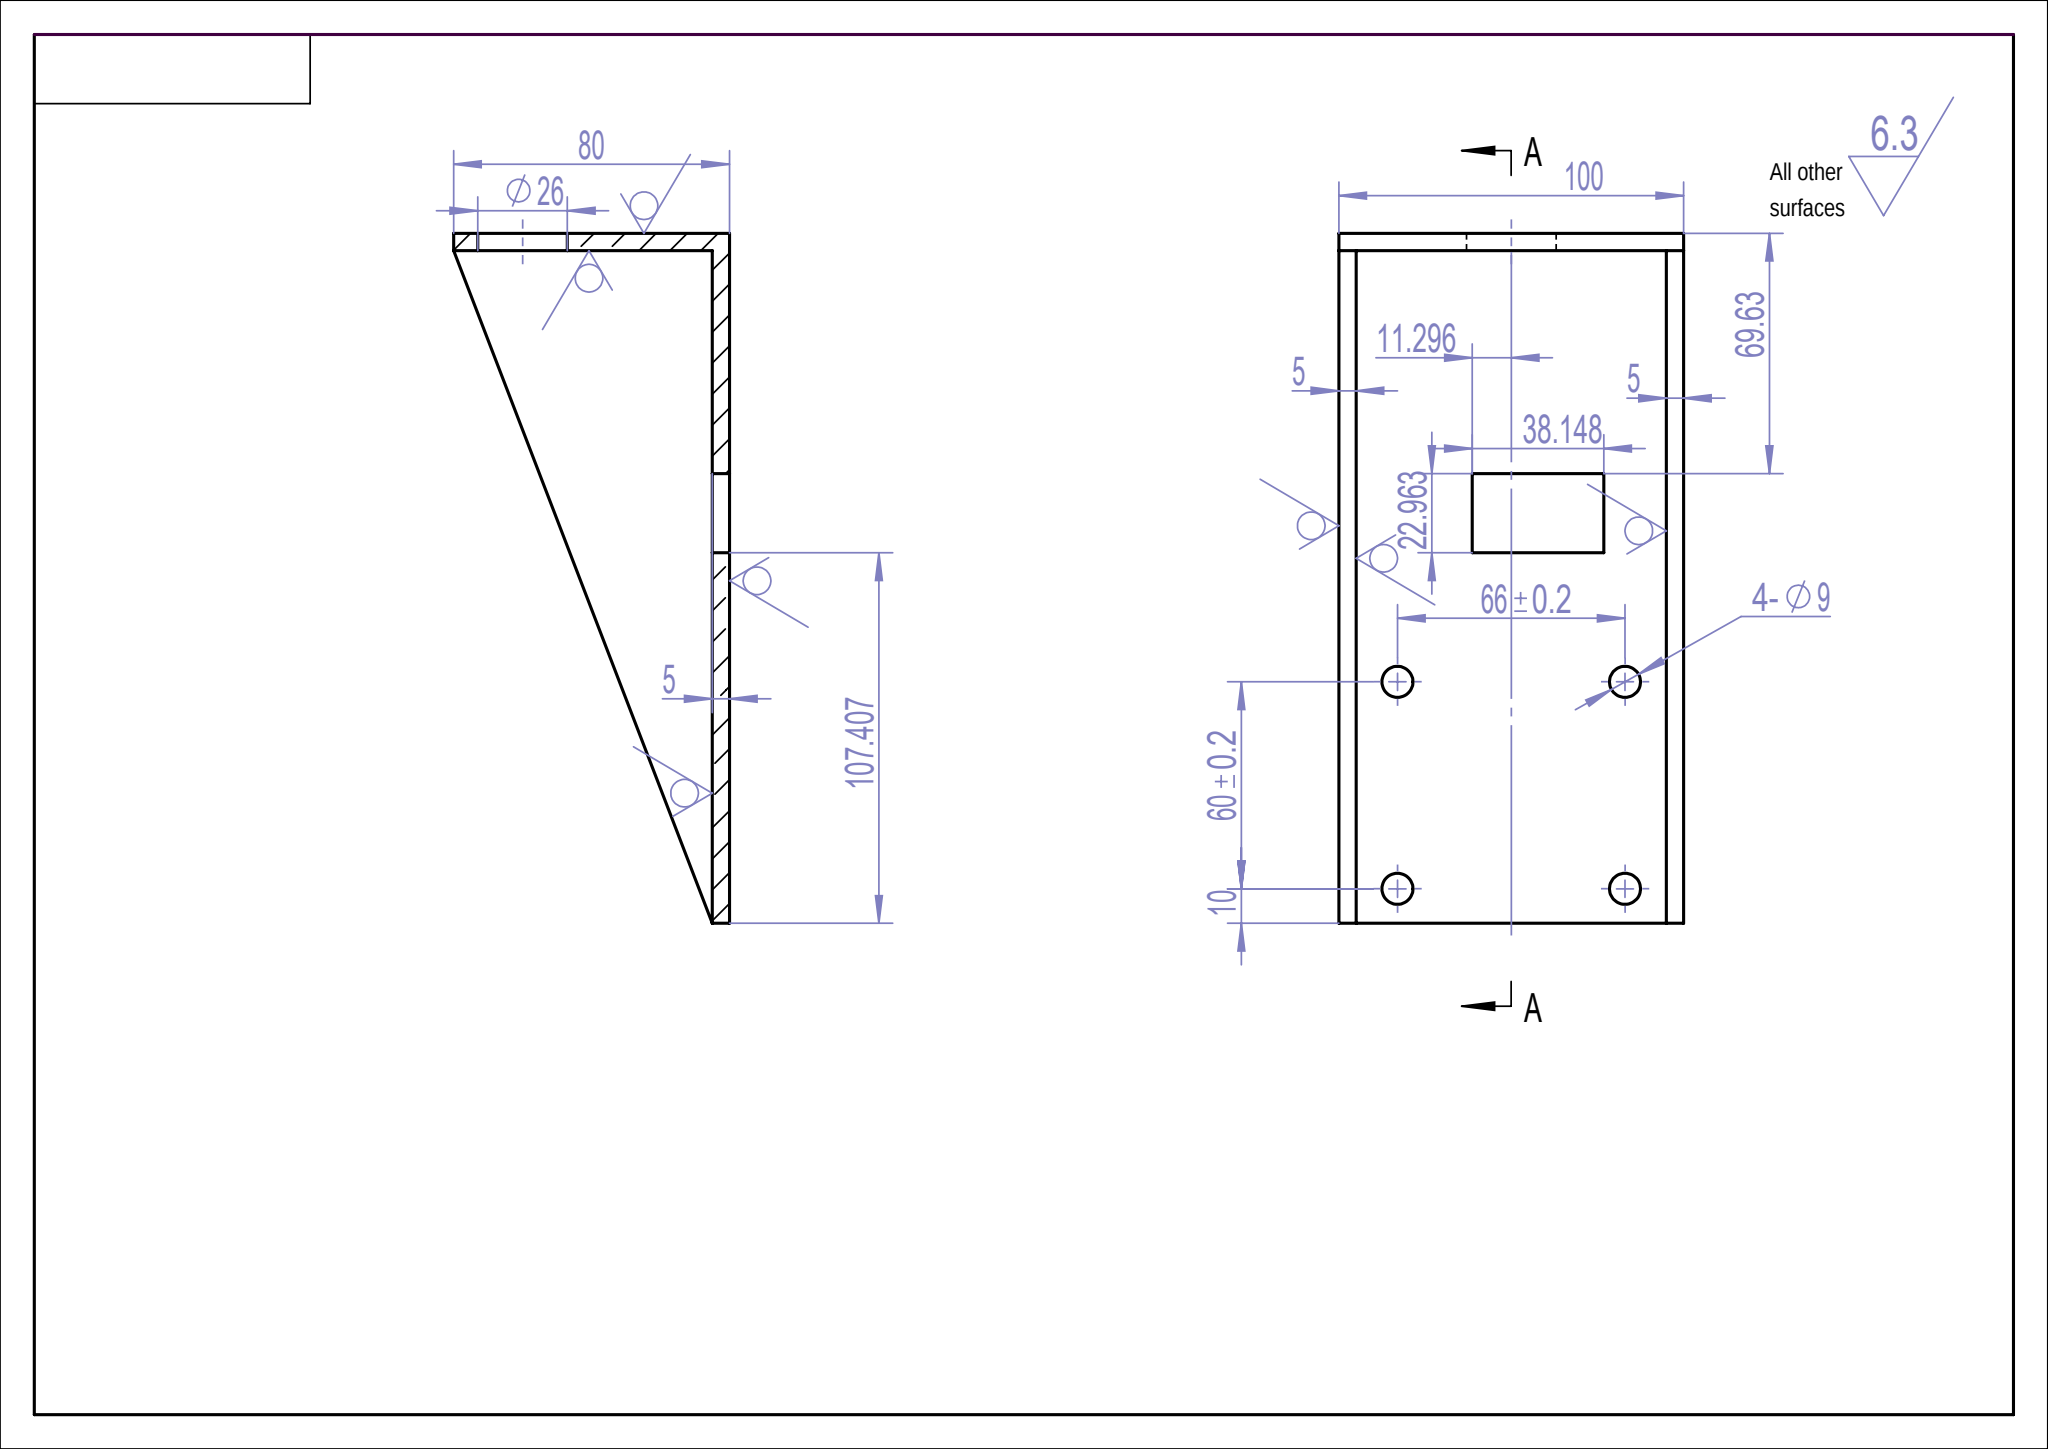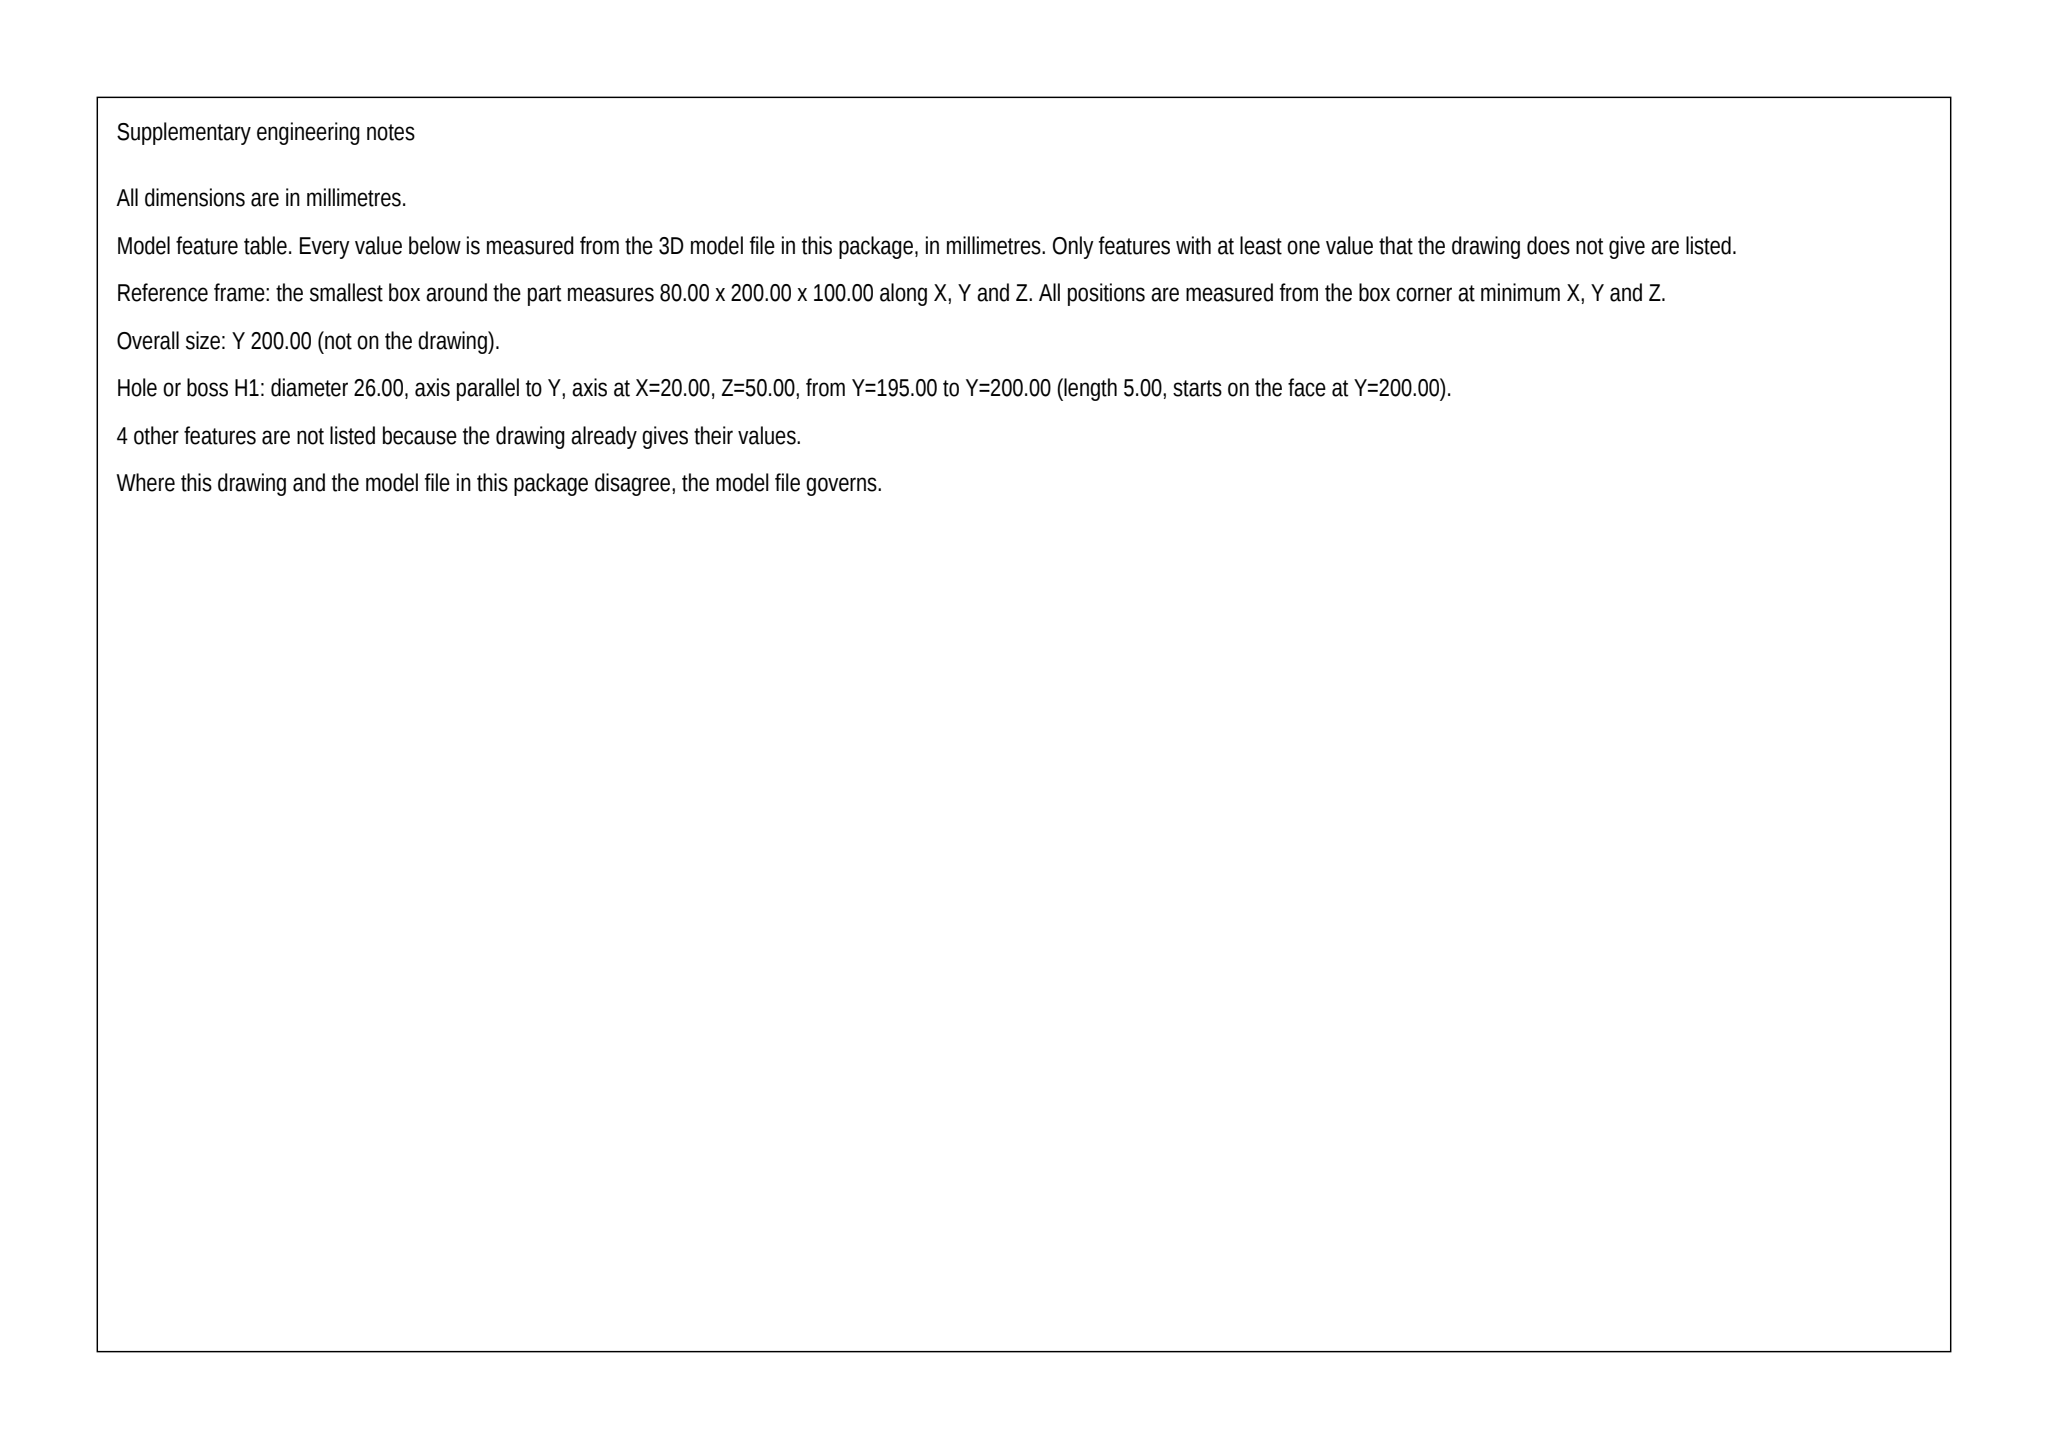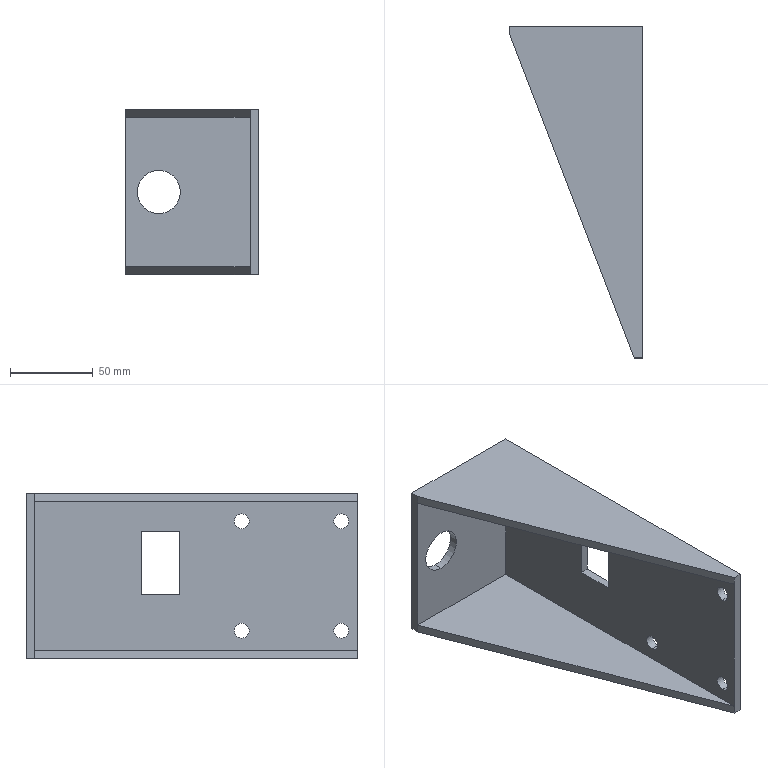Part | SolidWorks | mm | 1 solid | 26 faces | box 80 x 200 x 100 mm | volume 202318 mm3 | plane 16 | cylinder 10 | commonest cylinder face diameters 9 x8 26 x2
build123d program:
from build123d import *

# Parameters (mm, degrees)
BOSS_EXTRUDE1_DEPTH = 50
BOSS_EXTRUDE2_DEPTH = 5
SKETCH3_R           = 13
CUT_EXTRUDE1_DEPTH  = 5
SKETCH4_R           = 4.5
CUT_EXTRUDE2_DEPTH  = 5
SKETCH6_W           = 38.148
SKETCH6_H           = 22.963
CUT_EXTRUDE3_DEPTH  = 31


with BuildPart() as part:
    # Sketch1 → Boss-Extrude1 (new, symmetric)
    with BuildSketch(Plane.XY):
        Polygon((-48.173, 37.525), (31.827, 37.525), (31.827, -162.475), (26.827, -162.475), (26.827, 32.525), (-48.173, 32.525), align=None)
    extrude(amount=BOSS_EXTRUDE1_DEPTH, both=True)

    # Sketch2 → Boss-Extrude2 (add)
    with BuildSketch(Plane.XY.offset(50)):
        Polygon((-48.173, 32.525), (26.827, -162.475), (26.827, 32.525), align=None)
    boss_extrude2 = extrude(amount=-BOSS_EXTRUDE2_DEPTH)

    # Mirror1: Boss-Extrude2 across plane
    add(boss_extrude2.mirror(Plane.XY))

    # Sketch3 → Cut-Extrude1 (cut)
    with BuildSketch(Plane(origin=(0, 37.525, 0), x_dir=(1, 0, 0), z_dir=(0, 1, 0))):
        with Locations(Location((-28.173, 0, 0), (0, 0, 270))):
            Circle(SKETCH3_R)
    extrude(amount=-CUT_EXTRUDE1_DEPTH, mode=Mode.SUBTRACT)

    # Sketch4 → Cut-Extrude2 (cut)
    with BuildSketch(Plane.ZY.offset(-26.827)):
        with Locations((-33, -152.475)):
            Circle(SKETCH4_R)
        with Locations((33, -152.475)):
            Circle(SKETCH4_R)
        with Locations((-33, -92.475)):
            Circle(SKETCH4_R)
        with Locations((33, -92.475)):
            Circle(SKETCH4_R)
    extrude(amount=-CUT_EXTRUDE2_DEPTH, mode=Mode.SUBTRACT)

    # Sketch6 → Cut-Extrude3 (cut)
    with BuildSketch(Plane.ZY.offset(-26.827)):
        with Locations((7.778, -43.587)):
            Rectangle(SKETCH6_W, SKETCH6_H)
    extrude(amount=-CUT_EXTRUDE3_DEPTH, mode=Mode.SUBTRACT)


solid = part.part
STEP:
#1=CARTESIAN_POINT('',(31.827,-92.475,28.5));
#2=VERTEX_POINT('',#1);
#3=CARTESIAN_POINT('',(31.827,-92.475,37.5));
#4=VERTEX_POINT('',#3);
#5=CARTESIAN_POINT('',(31.827,-92.475,33.));
#6=DIRECTION('',(-1.,0.,0.));
#7=DIRECTION('',(0.,0.,1.));
#8=AXIS2_PLACEMENT_3D('',#5,#6,#7);
#9=CIRCLE('',#8,4.5);
#10=EDGE_CURVE('',#2,#4,#9,.T.);
#11=ORIENTED_EDGE('',*,*,#10,.F.);
#12=CARTESIAN_POINT('',(26.827,-92.475,28.5));
#13=VERTEX_POINT('',#12);
#14=CARTESIAN_POINT('',(31.827,-92.475,28.5));
#15=DIRECTION('',(-1.,0.,0.));
#16=VECTOR('',#15,1000.);
#17=LINE('',#14,#16);
#18=EDGE_CURVE('',#2,#13,#17,.T.);
#19=ORIENTED_EDGE('',*,*,#18,.T.);
#20=CARTESIAN_POINT('',(26.827,-92.475,37.5));
#21=VERTEX_POINT('',#20);
#22=CARTESIAN_POINT('',(26.827,-92.475,33.));
#23=DIRECTION('',(-1.,0.,0.));
#24=DIRECTION('',(0.,0.,1.));
#25=AXIS2_PLACEMENT_3D('',#22,#23,#24);
#26=CIRCLE('',#25,4.5);
#27=EDGE_CURVE('',#13,#21,#26,.T.);
#28=ORIENTED_EDGE('',*,*,#27,.T.);
#29=CARTESIAN_POINT('',(31.827,-92.475,37.5));
#30=DIRECTION('',(-1.,0.,0.));
#31=VECTOR('',#30,1000.);
#32=LINE('',#29,#31);
#33=EDGE_CURVE('',#4,#21,#32,.T.);
#34=ORIENTED_EDGE('',*,*,#33,.F.);
#35=EDGE_LOOP('',(#11,#19,#28,#34));
#36=FACE_OUTER_BOUND('',#35,.T.);
#37=CARTESIAN_POINT('',(31.827,-92.475,33.));
#38=DIRECTION('',(-1.,0.,0.));
#39=DIRECTION('',(0.,0.,1.));
#40=AXIS2_PLACEMENT_3D('',#37,#38,#39);
#41=CYLINDRICAL_SURFACE('',#40,4.5);
#42=ADVANCED_FACE('',(#36),#41,.F.);
#43=CARTESIAN_POINT('',(31.827,-92.475,-37.5));
#44=VERTEX_POINT('',#43);
#45=CARTESIAN_POINT('',(31.827,-92.475,-28.5));
#46=VERTEX_POINT('',#45);
#47=CARTESIAN_POINT('',(31.827,-92.475,-33.));
#48=DIRECTION('',(-1.,0.,0.));
#49=DIRECTION('',(0.,0.,1.));
#50=AXIS2_PLACEMENT_3D('',#47,#48,#49);
#51=CIRCLE('',#50,4.5);
#52=EDGE_CURVE('',#44,#46,#51,.T.);
#53=ORIENTED_EDGE('',*,*,#52,.F.);
#54=CARTESIAN_POINT('',(26.827,-92.475,-37.5));
#55=VERTEX_POINT('',#54);
#56=CARTESIAN_POINT('',(31.827,-92.475,-37.5));
#57=DIRECTION('',(-1.,0.,0.));
#58=VECTOR('',#57,1000.);
#59=LINE('',#56,#58);
#60=EDGE_CURVE('',#44,#55,#59,.T.);
#61=ORIENTED_EDGE('',*,*,#60,.T.);
#62=CARTESIAN_POINT('',(26.827,-92.475,-28.5));
#63=VERTEX_POINT('',#62);
#64=CARTESIAN_POINT('',(26.827,-92.475,-33.));
#65=DIRECTION('',(-1.,0.,0.));
#66=DIRECTION('',(0.,0.,1.));
#67=AXIS2_PLACEMENT_3D('',#64,#65,#66);
#68=CIRCLE('',#67,4.5);
#69=EDGE_CURVE('',#55,#63,#68,.T.);
#70=ORIENTED_EDGE('',*,*,#69,.T.);
#71=CARTESIAN_POINT('',(31.827,-92.475,-28.5));
#72=DIRECTION('',(-1.,0.,0.));
#73=VECTOR('',#72,1000.);
#74=LINE('',#71,#73);
#75=EDGE_CURVE('',#46,#63,#74,.T.);
#76=ORIENTED_EDGE('',*,*,#75,.F.);
#77=EDGE_LOOP('',(#53,#61,#70,#76));
#78=FACE_OUTER_BOUND('',#77,.T.);
#79=CARTESIAN_POINT('',(31.827,-92.475,-33.));
#80=DIRECTION('',(-1.,0.,0.));
#81=DIRECTION('',(0.,0.,1.));
#82=AXIS2_PLACEMENT_3D('',#79,#80,#81);
#83=CYLINDRICAL_SURFACE('',#82,4.5);
#84=ADVANCED_FACE('',(#78),#83,.F.);
#85=CARTESIAN_POINT('',(31.827,-152.475,28.5));
#86=VERTEX_POINT('',#85);
#87=CARTESIAN_POINT('',(31.827,-152.475,37.5));
#88=VERTEX_POINT('',#87);
#89=CARTESIAN_POINT('',(31.827,-152.475,33.));
#90=DIRECTION('',(-1.,0.,0.));
#91=DIRECTION('',(0.,0.,1.));
#92=AXIS2_PLACEMENT_3D('',#89,#90,#91);
#93=CIRCLE('',#92,4.5);
#94=EDGE_CURVE('',#86,#88,#93,.T.);
#95=ORIENTED_EDGE('',*,*,#94,.F.);
#96=CARTESIAN_POINT('',(26.827,-152.475,28.5));
#97=VERTEX_POINT('',#96);
#98=CARTESIAN_POINT('',(31.827,-152.475,28.5));
#99=DIRECTION('',(-1.,0.,0.));
#100=VECTOR('',#99,1000.);
#101=LINE('',#98,#100);
#102=EDGE_CURVE('',#86,#97,#101,.T.);
#103=ORIENTED_EDGE('',*,*,#102,.T.);
#104=CARTESIAN_POINT('',(26.827,-152.475,37.5));
#105=VERTEX_POINT('',#104);
#106=CARTESIAN_POINT('',(26.827,-152.475,33.));
#107=DIRECTION('',(-1.,0.,0.));
#108=DIRECTION('',(0.,0.,1.));
#109=AXIS2_PLACEMENT_3D('',#106,#107,#108);
#110=CIRCLE('',#109,4.5);
#111=EDGE_CURVE('',#97,#105,#110,.T.);
#112=ORIENTED_EDGE('',*,*,#111,.T.);
#113=CARTESIAN_POINT('',(31.827,-152.475,37.5));
#114=DIRECTION('',(-1.,0.,0.));
#115=VECTOR('',#114,1000.);
#116=LINE('',#113,#115);
#117=EDGE_CURVE('',#88,#105,#116,.T.);
#118=ORIENTED_EDGE('',*,*,#117,.F.);
#119=EDGE_LOOP('',(#95,#103,#112,#118));
#120=FACE_OUTER_BOUND('',#119,.T.);
#121=CARTESIAN_POINT('',(31.827,-152.475,33.));
#122=DIRECTION('',(-1.,0.,0.));
#123=DIRECTION('',(0.,0.,1.));
#124=AXIS2_PLACEMENT_3D('',#121,#122,#123);
#125=CYLINDRICAL_SURFACE('',#124,4.5);
#126=ADVANCED_FACE('',(#120),#125,.F.);
#127=CARTESIAN_POINT('',(31.827,-152.475,-37.5));
#128=VERTEX_POINT('',#127);
#129=CARTESIAN_POINT('',(31.827,-152.475,-28.5));
#130=VERTEX_POINT('',#129);
#131=CARTESIAN_POINT('',(31.827,-152.475,-33.));
#132=DIRECTION('',(-1.,0.,0.));
#133=DIRECTION('',(0.,0.,1.));
#134=AXIS2_PLACEMENT_3D('',#131,#132,#133);
#135=CIRCLE('',#134,4.5);
#136=EDGE_CURVE('',#128,#130,#135,.T.);
#137=ORIENTED_EDGE('',*,*,#136,.F.);
#138=CARTESIAN_POINT('',(26.827,-152.475,-37.5));
#139=VERTEX_POINT('',#138);
#140=CARTESIAN_POINT('',(31.827,-152.475,-37.5));
#141=DIRECTION('',(-1.,0.,0.));
#142=VECTOR('',#141,1000.);
#143=LINE('',#140,#142);
#144=EDGE_CURVE('',#128,#139,#143,.T.);
#145=ORIENTED_EDGE('',*,*,#144,.T.);
#146=CARTESIAN_POINT('',(26.827,-152.475,-28.5));
#147=VERTEX_POINT('',#146);
#148=CARTESIAN_POINT('',(26.827,-152.475,-33.));
#149=DIRECTION('',(-1.,0.,0.));
#150=DIRECTION('',(0.,0.,1.));
#151=AXIS2_PLACEMENT_3D('',#148,#149,#150);
#152=CIRCLE('',#151,4.5);
#153=EDGE_CURVE('',#139,#147,#152,.T.);
#154=ORIENTED_EDGE('',*,*,#153,.T.);
#155=CARTESIAN_POINT('',(31.827,-152.475,-28.5));
#156=DIRECTION('',(-1.,0.,0.));
#157=VECTOR('',#156,1000.);
#158=LINE('',#155,#157);
#159=EDGE_CURVE('',#130,#147,#158,.T.);
#160=ORIENTED_EDGE('',*,*,#159,.F.);
#161=EDGE_LOOP('',(#137,#145,#154,#160));
#162=FACE_OUTER_BOUND('',#161,.T.);
#163=CARTESIAN_POINT('',(31.827,-152.475,-33.));
#164=DIRECTION('',(-1.,0.,0.));
#165=DIRECTION('',(0.,0.,1.));
#166=AXIS2_PLACEMENT_3D('',#163,#164,#165);
#167=CYLINDRICAL_SURFACE('',#166,4.5);
#168=ADVANCED_FACE('',(#162),#167,.F.);
#169=CARTESIAN_POINT('',(-28.173,32.525,-13.));
#170=VERTEX_POINT('',#169);
#171=CARTESIAN_POINT('',(-28.173,32.525,13.));
#172=VERTEX_POINT('',#171);
#173=CARTESIAN_POINT('',(-28.173,32.525,0.));
#174=DIRECTION('',(0.,1.,0.));
#175=DIRECTION('',(0.,0.,1.));
#176=AXIS2_PLACEMENT_3D('',#173,#174,#175);
#177=CIRCLE('',#176,13.);
#178=EDGE_CURVE('',#170,#172,#177,.T.);
#179=ORIENTED_EDGE('',*,*,#178,.F.);
#180=CARTESIAN_POINT('',(-28.173,37.525,-13.));
#181=VERTEX_POINT('',#180);
#182=CARTESIAN_POINT('',(-28.173,32.525,-13.));
#183=DIRECTION('',(0.,1.,0.));
#184=VECTOR('',#183,1000.);
#185=LINE('',#182,#184);
#186=EDGE_CURVE('',#170,#181,#185,.T.);
#187=ORIENTED_EDGE('',*,*,#186,.T.);
#188=CARTESIAN_POINT('',(-28.173,37.525,13.));
#189=VERTEX_POINT('',#188);
#190=CARTESIAN_POINT('',(-28.173,37.525,0.));
#191=DIRECTION('',(0.,1.,0.));
#192=DIRECTION('',(0.,0.,1.));
#193=AXIS2_PLACEMENT_3D('',#190,#191,#192);
#194=CIRCLE('',#193,13.);
#195=EDGE_CURVE('',#181,#189,#194,.T.);
#196=ORIENTED_EDGE('',*,*,#195,.T.);
#197=CARTESIAN_POINT('',(-28.173,32.525,13.));
#198=DIRECTION('',(0.,1.,0.));
#199=VECTOR('',#198,1000.);
#200=LINE('',#197,#199);
#201=EDGE_CURVE('',#172,#189,#200,.T.);
#202=ORIENTED_EDGE('',*,*,#201,.F.);
#203=EDGE_LOOP('',(#179,#187,#196,#202));
#204=FACE_OUTER_BOUND('',#203,.T.);
#205=CARTESIAN_POINT('',(-28.173,32.525,0.));
#206=DIRECTION('',(0.,1.,0.));
#207=DIRECTION('',(0.,0.,1.));
#208=AXIS2_PLACEMENT_3D('',#205,#206,#207);
#209=CYLINDRICAL_SURFACE('',#208,13.);
#210=ADVANCED_FACE('',(#204),#209,.F.);
#211=CARTESIAN_POINT('',(-48.173,37.525,-50.));
#212=VERTEX_POINT('',#211);
#213=CARTESIAN_POINT('',(-48.173,32.525,-50.));
#214=VERTEX_POINT('',#213);
#215=CARTESIAN_POINT('',(-48.173,37.525,-50.));
#216=DIRECTION('',(0.,-1.,0.));
#217=VECTOR('',#216,1000.);
#218=LINE('',#215,#217);
#219=EDGE_CURVE('',#212,#214,#218,.T.);
#220=ORIENTED_EDGE('',*,*,#219,.T.);
#221=CARTESIAN_POINT('',(-48.173,32.525,-45.));
#222=VERTEX_POINT('',#221);
#223=CARTESIAN_POINT('',(-48.173,32.525,-45.));
#224=DIRECTION('',(0.,0.,-1.));
#225=VECTOR('',#224,1000.);
#226=LINE('',#223,#225);
#227=EDGE_CURVE('',#222,#214,#226,.T.);
#228=ORIENTED_EDGE('',*,*,#227,.F.);
#229=CARTESIAN_POINT('',(-48.173,32.525,45.));
#230=VERTEX_POINT('',#229);
#231=CARTESIAN_POINT('',(-48.173,32.525,50.));
#232=DIRECTION('',(0.,0.,-1.));
#233=VECTOR('',#232,1000.);
#234=LINE('',#231,#233);
#235=EDGE_CURVE('',#230,#222,#234,.T.);
#236=ORIENTED_EDGE('',*,*,#235,.F.);
#237=CARTESIAN_POINT('',(-48.173,32.525,50.));
#238=VERTEX_POINT('',#237);
#239=CARTESIAN_POINT('',(-48.173,32.525,50.));
#240=DIRECTION('',(0.,0.,-1.));
#241=VECTOR('',#240,1000.);
#242=LINE('',#239,#241);
#243=EDGE_CURVE('',#238,#230,#242,.T.);
#244=ORIENTED_EDGE('',*,*,#243,.F.);
#245=CARTESIAN_POINT('',(-48.173,37.525,50.));
#246=VERTEX_POINT('',#245);
#247=CARTESIAN_POINT('',(-48.173,37.525,50.));
#248=DIRECTION('',(0.,-1.,0.));
#249=VECTOR('',#248,1000.);
#250=LINE('',#247,#249);
#251=EDGE_CURVE('',#246,#238,#250,.T.);
#252=ORIENTED_EDGE('',*,*,#251,.F.);
#253=CARTESIAN_POINT('',(-48.173,37.525,50.));
#254=DIRECTION('',(0.,0.,-1.));
#255=VECTOR('',#254,1000.);
#256=LINE('',#253,#255);
#257=EDGE_CURVE('',#246,#212,#256,.T.);
#258=ORIENTED_EDGE('',*,*,#257,.T.);
#259=EDGE_LOOP('',(#220,#228,#236,#244,#252,#258));
#260=FACE_OUTER_BOUND('',#259,.T.);
#261=CARTESIAN_POINT('',(-48.173,37.525,50.));
#262=DIRECTION('',(1.,0.,0.));
#263=DIRECTION('',(0.,0.,-1.));
#264=AXIS2_PLACEMENT_3D('',#261,#262,#263);
#265=PLANE('',#264);
#266=ADVANCED_FACE('',(#260),#265,.F.);
#267=CARTESIAN_POINT('',(-28.173,32.525,0.));
#268=DIRECTION('',(0.,1.,0.));
#269=DIRECTION('',(0.,0.,1.));
#270=AXIS2_PLACEMENT_3D('',#267,#268,#269);
#271=CIRCLE('',#270,13.);
#272=EDGE_CURVE('',#172,#170,#271,.T.);
#273=ORIENTED_EDGE('',*,*,#272,.T.);
#274=ORIENTED_EDGE('',*,*,#178,.T.);
#275=EDGE_LOOP('',(#273,#274));
#276=FACE_BOUND('',#275,.T.);
#277=ORIENTED_EDGE('',*,*,#235,.T.);
#278=CARTESIAN_POINT('',(26.827,32.525,-45.));
#279=VERTEX_POINT('',#278);
#280=CARTESIAN_POINT('',(26.827,32.525,-45.));
#281=DIRECTION('',(-1.,0.,0.));
#282=VECTOR('',#281,1000.);
#283=LINE('',#280,#282);
#284=EDGE_CURVE('',#279,#222,#283,.T.);
#285=ORIENTED_EDGE('',*,*,#284,.F.);
#286=CARTESIAN_POINT('',(26.827,32.525,45.));
#287=VERTEX_POINT('',#286);
#288=CARTESIAN_POINT('',(26.827,32.525,50.));
#289=DIRECTION('',(0.,0.,-1.));
#290=VECTOR('',#289,1000.);
#291=LINE('',#288,#290);
#292=EDGE_CURVE('',#287,#279,#291,.T.);
#293=ORIENTED_EDGE('',*,*,#292,.F.);
#294=CARTESIAN_POINT('',(26.827,32.525,45.));
#295=DIRECTION('',(-1.,0.,0.));
#296=VECTOR('',#295,1000.);
#297=LINE('',#294,#296);
#298=EDGE_CURVE('',#287,#230,#297,.T.);
#299=ORIENTED_EDGE('',*,*,#298,.T.);
#300=EDGE_LOOP('',(#277,#285,#293,#299));
#301=FACE_OUTER_BOUND('',#300,.T.);
#302=CARTESIAN_POINT('',(-48.173,32.525,50.));
#303=DIRECTION('',(0.,1.,0.));
#304=DIRECTION('',(0.,0.,1.));
#305=AXIS2_PLACEMENT_3D('',#302,#303,#304);
#306=PLANE('',#305);
#307=ADVANCED_FACE('',(#276,#301),#306,.F.);
#308=CARTESIAN_POINT('',(26.827,-55.068,-11.296));
#309=VERTEX_POINT('',#308);
#310=CARTESIAN_POINT('',(26.827,-55.068,26.852));
#311=VERTEX_POINT('',#310);
#312=CARTESIAN_POINT('',(26.827,-55.068,-11.296));
#313=DIRECTION('',(0.,0.,1.));
#314=VECTOR('',#313,1000.);
#315=LINE('',#312,#314);
#316=EDGE_CURVE('',#309,#311,#315,.T.);
#317=ORIENTED_EDGE('',*,*,#316,.F.);
#318=CARTESIAN_POINT('',(26.827,-32.105,-11.296));
#319=VERTEX_POINT('',#318);
#320=CARTESIAN_POINT('',(26.827,-32.105,-11.296));
#321=DIRECTION('',(0.,-1.,0.));
#322=VECTOR('',#321,1000.);
#323=LINE('',#320,#322);
#324=EDGE_CURVE('',#319,#309,#323,.T.);
#325=ORIENTED_EDGE('',*,*,#324,.F.);
#326=CARTESIAN_POINT('',(26.827,-32.105,26.852));
#327=VERTEX_POINT('',#326);
#328=CARTESIAN_POINT('',(26.827,-32.105,-11.296));
#329=DIRECTION('',(0.,0.,-1.));
#330=VECTOR('',#329,1000.);
#331=LINE('',#328,#330);
#332=EDGE_CURVE('',#327,#319,#331,.T.);
#333=ORIENTED_EDGE('',*,*,#332,.F.);
#334=CARTESIAN_POINT('',(26.827,-32.105,26.852));
#335=DIRECTION('',(0.,1.,0.));
#336=VECTOR('',#335,1000.);
#337=LINE('',#334,#336);
#338=EDGE_CURVE('',#311,#327,#337,.T.);
#339=ORIENTED_EDGE('',*,*,#338,.F.);
#340=EDGE_LOOP('',(#317,#325,#333,#339));
#341=FACE_BOUND('',#340,.T.);
#342=CARTESIAN_POINT('',(26.827,-92.475,33.));
#343=DIRECTION('',(-1.,0.,0.));
#344=DIRECTION('',(0.,0.,1.));
#345=AXIS2_PLACEMENT_3D('',#342,#343,#344);
#346=CIRCLE('',#345,4.5);
#347=EDGE_CURVE('',#21,#13,#346,.T.);
#348=ORIENTED_EDGE('',*,*,#347,.F.);
#349=ORIENTED_EDGE('',*,*,#27,.F.);
#350=EDGE_LOOP('',(#348,#349));
#351=FACE_BOUND('',#350,.T.);
#352=CARTESIAN_POINT('',(26.827,-92.475,-33.));
#353=DIRECTION('',(-1.,0.,0.));
#354=DIRECTION('',(0.,0.,1.));
#355=AXIS2_PLACEMENT_3D('',#352,#353,#354);
#356=CIRCLE('',#355,4.5);
#357=EDGE_CURVE('',#63,#55,#356,.T.);
#358=ORIENTED_EDGE('',*,*,#357,.F.);
#359=ORIENTED_EDGE('',*,*,#69,.F.);
#360=EDGE_LOOP('',(#358,#359));
#361=FACE_BOUND('',#360,.T.);
#362=CARTESIAN_POINT('',(26.827,-152.475,33.));
#363=DIRECTION('',(-1.,0.,0.));
#364=DIRECTION('',(0.,0.,1.));
#365=AXIS2_PLACEMENT_3D('',#362,#363,#364);
#366=CIRCLE('',#365,4.5);
#367=EDGE_CURVE('',#105,#97,#366,.T.);
#368=ORIENTED_EDGE('',*,*,#367,.F.);
#369=ORIENTED_EDGE('',*,*,#111,.F.);
#370=EDGE_LOOP('',(#368,#369));
#371=FACE_BOUND('',#370,.T.);
#372=CARTESIAN_POINT('',(26.827,-152.475,-33.));
#373=DIRECTION('',(-1.,0.,0.));
#374=DIRECTION('',(0.,0.,1.));
#375=AXIS2_PLACEMENT_3D('',#372,#373,#374);
#376=CIRCLE('',#375,4.5);
#377=EDGE_CURVE('',#147,#139,#376,.T.);
#378=ORIENTED_EDGE('',*,*,#377,.F.);
#379=ORIENTED_EDGE('',*,*,#153,.F.);
#380=EDGE_LOOP('',(#378,#379));
#381=FACE_BOUND('',#380,.T.);
#382=ORIENTED_EDGE('',*,*,#292,.T.);
#383=CARTESIAN_POINT('',(26.827,-162.475,-45.));
#384=VERTEX_POINT('',#383);
#385=CARTESIAN_POINT('',(26.827,-162.475,-45.));
#386=DIRECTION('',(0.,1.,0.));
#387=VECTOR('',#386,1000.);
#388=LINE('',#385,#387);
#389=EDGE_CURVE('',#384,#279,#388,.T.);
#390=ORIENTED_EDGE('',*,*,#389,.F.);
#391=CARTESIAN_POINT('',(26.827,-162.475,45.));
#392=VERTEX_POINT('',#391);
#393=CARTESIAN_POINT('',(26.827,-162.475,50.));
#394=DIRECTION('',(0.,0.,-1.));
#395=VECTOR('',#394,1000.);
#396=LINE('',#393,#395);
#397=EDGE_CURVE('',#392,#384,#396,.T.);
#398=ORIENTED_EDGE('',*,*,#397,.F.);
#399=CARTESIAN_POINT('',(26.827,-162.475,45.));
#400=DIRECTION('',(0.,1.,0.));
#401=VECTOR('',#400,1000.);
#402=LINE('',#399,#401);
#403=EDGE_CURVE('',#392,#287,#402,.T.);
#404=ORIENTED_EDGE('',*,*,#403,.T.);
#405=EDGE_LOOP('',(#382,#390,#398,#404));
#406=FACE_OUTER_BOUND('',#405,.T.);
#407=CARTESIAN_POINT('',(26.827,32.525,50.));
#408=DIRECTION('',(1.,0.,0.));
#409=DIRECTION('',(0.,0.,-1.));
#410=AXIS2_PLACEMENT_3D('',#407,#408,#409);
#411=PLANE('',#410);
#412=ADVANCED_FACE('',(#341,#351,#361,#371,#381,#406),#411,.F.);
#413=CARTESIAN_POINT('',(26.827,-162.475,-50.));
#414=VERTEX_POINT('',#413);
#415=CARTESIAN_POINT('',(31.827,-162.475,-50.));
#416=VERTEX_POINT('',#415);
#417=CARTESIAN_POINT('',(26.827,-162.475,-50.));
#418=DIRECTION('',(1.,0.,0.));
#419=VECTOR('',#418,1000.);
#420=LINE('',#417,#419);
#421=EDGE_CURVE('',#414,#416,#420,.T.);
#422=ORIENTED_EDGE('',*,*,#421,.T.);
#423=CARTESIAN_POINT('',(31.827,-162.475,50.));
#424=VERTEX_POINT('',#423);
#425=CARTESIAN_POINT('',(31.827,-162.475,50.));
#426=DIRECTION('',(0.,0.,-1.));
#427=VECTOR('',#426,1000.);
#428=LINE('',#425,#427);
#429=EDGE_CURVE('',#424,#416,#428,.T.);
#430=ORIENTED_EDGE('',*,*,#429,.F.);
#431=CARTESIAN_POINT('',(26.827,-162.475,50.));
#432=VERTEX_POINT('',#431);
#433=CARTESIAN_POINT('',(26.827,-162.475,50.));
#434=DIRECTION('',(1.,0.,0.));
#435=VECTOR('',#434,1000.);
#436=LINE('',#433,#435);
#437=EDGE_CURVE('',#432,#424,#436,.T.);
#438=ORIENTED_EDGE('',*,*,#437,.F.);
#439=CARTESIAN_POINT('',(26.827,-162.475,50.));
#440=DIRECTION('',(0.,0.,-1.));
#441=VECTOR('',#440,1000.);
#442=LINE('',#439,#441);
#443=EDGE_CURVE('',#432,#392,#442,.T.);
#444=ORIENTED_EDGE('',*,*,#443,.T.);
#445=ORIENTED_EDGE('',*,*,#397,.T.);
#446=CARTESIAN_POINT('',(26.827,-162.475,-45.));
#447=DIRECTION('',(0.,0.,-1.));
#448=VECTOR('',#447,1000.);
#449=LINE('',#446,#448);
#450=EDGE_CURVE('',#384,#414,#449,.T.);
#451=ORIENTED_EDGE('',*,*,#450,.T.);
#452=EDGE_LOOP('',(#422,#430,#438,#444,#445,#451));
#453=FACE_OUTER_BOUND('',#452,.T.);
#454=CARTESIAN_POINT('',(26.827,-162.475,50.));
#455=DIRECTION('',(0.,1.,0.));
#456=DIRECTION('',(0.,0.,1.));
#457=AXIS2_PLACEMENT_3D('',#454,#455,#456);
#458=PLANE('',#457);
#459=ADVANCED_FACE('',(#453),#458,.F.);
#460=CARTESIAN_POINT('',(31.827,-32.105,26.852));
#461=VERTEX_POINT('',#460);
#462=CARTESIAN_POINT('',(31.827,-32.105,-11.296));
#463=VERTEX_POINT('',#462);
#464=CARTESIAN_POINT('',(31.827,-32.105,50.));
#465=DIRECTION('',(0.,0.,-1.));
#466=VECTOR('',#465,1000.);
#467=LINE('',#464,#466);
#468=EDGE_CURVE('',#461,#463,#467,.T.);
#469=ORIENTED_EDGE('',*,*,#468,.T.);
#470=CARTESIAN_POINT('',(31.827,-55.068,-11.296));
#471=VERTEX_POINT('',#470);
#472=CARTESIAN_POINT('',(31.827,37.525,-11.296));
#473=DIRECTION('',(0.,-1.,0.));
#474=VECTOR('',#473,1000.);
#475=LINE('',#472,#474);
#476=EDGE_CURVE('',#463,#471,#475,.T.);
#477=ORIENTED_EDGE('',*,*,#476,.T.);
#478=CARTESIAN_POINT('',(31.827,-55.068,26.852));
#479=VERTEX_POINT('',#478);
#480=CARTESIAN_POINT('',(31.827,-55.068,50.));
#481=DIRECTION('',(0.,0.,1.));
#482=VECTOR('',#481,1000.);
#483=LINE('',#480,#482);
#484=EDGE_CURVE('',#471,#479,#483,.T.);
#485=ORIENTED_EDGE('',*,*,#484,.T.);
#486=CARTESIAN_POINT('',(31.827,37.525,26.852));
#487=DIRECTION('',(-0.,1.,0.));
#488=VECTOR('',#487,1000.);
#489=LINE('',#486,#488);
#490=EDGE_CURVE('',#479,#461,#489,.T.);
#491=ORIENTED_EDGE('',*,*,#490,.T.);
#492=EDGE_LOOP('',(#469,#477,#485,#491));
#493=FACE_BOUND('',#492,.T.);
#494=CARTESIAN_POINT('',(31.827,-92.475,33.));
#495=DIRECTION('',(-1.,0.,0.));
#496=DIRECTION('',(0.,0.,1.));
#497=AXIS2_PLACEMENT_3D('',#494,#495,#496);
#498=CIRCLE('',#497,4.5);
#499=EDGE_CURVE('',#4,#2,#498,.T.);
#500=ORIENTED_EDGE('',*,*,#499,.T.);
#501=ORIENTED_EDGE('',*,*,#10,.T.);
#502=EDGE_LOOP('',(#500,#501));
#503=FACE_BOUND('',#502,.T.);
#504=CARTESIAN_POINT('',(31.827,-92.475,-33.));
#505=DIRECTION('',(-1.,0.,0.));
#506=DIRECTION('',(0.,0.,1.));
#507=AXIS2_PLACEMENT_3D('',#504,#505,#506);
#508=CIRCLE('',#507,4.5);
#509=EDGE_CURVE('',#46,#44,#508,.T.);
#510=ORIENTED_EDGE('',*,*,#509,.T.);
#511=ORIENTED_EDGE('',*,*,#52,.T.);
#512=EDGE_LOOP('',(#510,#511));
#513=FACE_BOUND('',#512,.T.);
#514=CARTESIAN_POINT('',(31.827,-152.475,33.));
#515=DIRECTION('',(-1.,0.,0.));
#516=DIRECTION('',(0.,0.,1.));
#517=AXIS2_PLACEMENT_3D('',#514,#515,#516);
#518=CIRCLE('',#517,4.5);
#519=EDGE_CURVE('',#88,#86,#518,.T.);
#520=ORIENTED_EDGE('',*,*,#519,.T.);
#521=ORIENTED_EDGE('',*,*,#94,.T.);
#522=EDGE_LOOP('',(#520,#521));
#523=FACE_BOUND('',#522,.T.);
#524=CARTESIAN_POINT('',(31.827,-152.475,-33.));
#525=DIRECTION('',(-1.,0.,0.));
#526=DIRECTION('',(0.,0.,1.));
#527=AXIS2_PLACEMENT_3D('',#524,#525,#526);
#528=CIRCLE('',#527,4.5);
#529=EDGE_CURVE('',#130,#128,#528,.T.);
#530=ORIENTED_EDGE('',*,*,#529,.T.);
#531=ORIENTED_EDGE('',*,*,#136,.T.);
#532=EDGE_LOOP('',(#530,#531));
#533=FACE_BOUND('',#532,.T.);
#534=CARTESIAN_POINT('',(31.827,37.525,-50.));
#535=VERTEX_POINT('',#534);
#536=CARTESIAN_POINT('',(31.827,37.525,-50.));
#537=DIRECTION('',(-0.,1.,0.));
#538=VECTOR('',#537,1000.);
#539=LINE('',#536,#538);
#540=EDGE_CURVE('',#416,#535,#539,.T.);
#541=ORIENTED_EDGE('',*,*,#540,.T.);
#542=CARTESIAN_POINT('',(31.827,37.525,50.));
#543=VERTEX_POINT('',#542);
#544=CARTESIAN_POINT('',(31.827,37.525,50.));
#545=DIRECTION('',(0.,0.,-1.));
#546=VECTOR('',#545,1000.);
#547=LINE('',#544,#546);
#548=EDGE_CURVE('',#543,#535,#547,.T.);
#549=ORIENTED_EDGE('',*,*,#548,.F.);
#550=CARTESIAN_POINT('',(31.827,37.525,50.));
#551=DIRECTION('',(-0.,1.,0.));
#552=VECTOR('',#551,1000.);
#553=LINE('',#550,#552);
#554=EDGE_CURVE('',#424,#543,#553,.T.);
#555=ORIENTED_EDGE('',*,*,#554,.F.);
#556=ORIENTED_EDGE('',*,*,#429,.T.);
#557=EDGE_LOOP('',(#541,#549,#555,#556));
#558=FACE_OUTER_BOUND('',#557,.T.);
#559=CARTESIAN_POINT('',(31.827,37.525,50.));
#560=DIRECTION('',(-1.,-0.,0.));
#561=DIRECTION('',(0.,-1.,0.));
#562=AXIS2_PLACEMENT_3D('',#559,#560,#561);
#563=PLANE('',#562);
#564=ADVANCED_FACE('',(#493,#503,#513,#523,#533,#558),#563,.F.);
#565=CARTESIAN_POINT('',(-28.173,37.525,0.));
#566=DIRECTION('',(0.,1.,0.));
#567=DIRECTION('',(0.,0.,1.));
#568=AXIS2_PLACEMENT_3D('',#565,#566,#567);
#569=CIRCLE('',#568,13.);
#570=EDGE_CURVE('',#189,#181,#569,.T.);
#571=ORIENTED_EDGE('',*,*,#570,.F.);
#572=ORIENTED_EDGE('',*,*,#195,.F.);
#573=EDGE_LOOP('',(#571,#572));
#574=FACE_BOUND('',#573,.T.);
#575=CARTESIAN_POINT('',(-48.173,37.525,-50.));
#576=DIRECTION('',(-1.,0.,0.));
#577=VECTOR('',#576,1000.);
#578=LINE('',#575,#577);
#579=EDGE_CURVE('',#535,#212,#578,.T.);
#580=ORIENTED_EDGE('',*,*,#579,.T.);
#581=ORIENTED_EDGE('',*,*,#257,.F.);
#582=CARTESIAN_POINT('',(-48.173,37.525,50.));
#583=DIRECTION('',(-1.,0.,0.));
#584=VECTOR('',#583,1000.);
#585=LINE('',#582,#584);
#586=EDGE_CURVE('',#543,#246,#585,.T.);
#587=ORIENTED_EDGE('',*,*,#586,.F.);
#588=ORIENTED_EDGE('',*,*,#548,.T.);
#589=EDGE_LOOP('',(#580,#581,#587,#588));
#590=FACE_OUTER_BOUND('',#589,.T.);
#591=CARTESIAN_POINT('',(-48.173,37.525,50.));
#592=DIRECTION('',(0.,-1.,0.));
#593=DIRECTION('',(0.,0.,-1.));
#594=AXIS2_PLACEMENT_3D('',#591,#592,#593);
#595=PLANE('',#594);
#596=ADVANCED_FACE('',(#574,#590),#595,.F.);
#597=ORIENTED_EDGE('',*,*,#251,.T.);
#598=CARTESIAN_POINT('',(-48.173,32.525,50.));
#599=DIRECTION('',(0.359,-0.9333,0.));
#600=VECTOR('',#599,1000.);
#601=LINE('',#598,#600);
#602=EDGE_CURVE('',#238,#432,#601,.T.);
#603=ORIENTED_EDGE('',*,*,#602,.T.);
#604=ORIENTED_EDGE('',*,*,#437,.T.);
#605=ORIENTED_EDGE('',*,*,#554,.T.);
#606=ORIENTED_EDGE('',*,*,#586,.T.);
#607=EDGE_LOOP('',(#597,#603,#604,#605,#606));
#608=FACE_OUTER_BOUND('',#607,.T.);
#609=CARTESIAN_POINT('',(0.,0.,50.));
#610=DIRECTION('',(0.,0.,1.));
#611=DIRECTION('',(1.,0.,0.));
#612=AXIS2_PLACEMENT_3D('',#609,#610,#611);
#613=PLANE('',#612);
#614=ADVANCED_FACE('',(#608),#613,.T.);
#615=ORIENTED_EDGE('',*,*,#219,.F.);
#616=ORIENTED_EDGE('',*,*,#579,.F.);
#617=ORIENTED_EDGE('',*,*,#540,.F.);
#618=ORIENTED_EDGE('',*,*,#421,.F.);
#619=CARTESIAN_POINT('',(-48.173,32.525,-50.));
#620=DIRECTION('',(0.359,-0.9333,0.));
#621=VECTOR('',#620,1000.);
#622=LINE('',#619,#621);
#623=EDGE_CURVE('',#214,#414,#622,.T.);
#624=ORIENTED_EDGE('',*,*,#623,.F.);
#625=EDGE_LOOP('',(#615,#616,#617,#618,#624));
#626=FACE_OUTER_BOUND('',#625,.T.);
#627=CARTESIAN_POINT('',(0.,0.,-50.));
#628=DIRECTION('',(0.,0.,1.));
#629=DIRECTION('',(1.,0.,0.));
#630=AXIS2_PLACEMENT_3D('',#627,#628,#629);
#631=PLANE('',#630);
#632=ADVANCED_FACE('',(#626),#631,.F.);
#633=ORIENTED_EDGE('',*,*,#602,.F.);
#634=ORIENTED_EDGE('',*,*,#243,.T.);
#635=CARTESIAN_POINT('',(-48.173,32.525,45.));
#636=DIRECTION('',(0.359,-0.9333,0.));
#637=VECTOR('',#636,1000.);
#638=LINE('',#635,#637);
#639=EDGE_CURVE('',#230,#392,#638,.T.);
#640=ORIENTED_EDGE('',*,*,#639,.T.);
#641=ORIENTED_EDGE('',*,*,#443,.F.);
#642=EDGE_LOOP('',(#633,#634,#640,#641));
#643=FACE_OUTER_BOUND('',#642,.T.);
#644=CARTESIAN_POINT('',(-48.173,32.525,45.));
#645=DIRECTION('',(-0.9333,-0.359,0.));
#646=DIRECTION('',(0.359,-0.9333,0.));
#647=AXIS2_PLACEMENT_3D('',#644,#645,#646);
#648=PLANE('',#647);
#649=ADVANCED_FACE('',(#643),#648,.T.);
#650=ORIENTED_EDGE('',*,*,#298,.F.);
#651=ORIENTED_EDGE('',*,*,#403,.F.);
#652=ORIENTED_EDGE('',*,*,#639,.F.);
#653=EDGE_LOOP('',(#650,#651,#652));
#654=FACE_OUTER_BOUND('',#653,.T.);
#655=CARTESIAN_POINT('',(0.,0.,45.));
#656=DIRECTION('',(0.,0.,-1.));
#657=DIRECTION('',(-1.,0.,0.));
#658=AXIS2_PLACEMENT_3D('',#655,#656,#657);
#659=PLANE('',#658);
#660=ADVANCED_FACE('',(#654),#659,.T.);
#661=ORIENTED_EDGE('',*,*,#623,.T.);
#662=ORIENTED_EDGE('',*,*,#450,.F.);
#663=CARTESIAN_POINT('',(-48.173,32.525,-45.));
#664=DIRECTION('',(0.359,-0.9333,0.));
#665=VECTOR('',#664,1000.);
#666=LINE('',#663,#665);
#667=EDGE_CURVE('',#222,#384,#666,.T.);
#668=ORIENTED_EDGE('',*,*,#667,.F.);
#669=ORIENTED_EDGE('',*,*,#227,.T.);
#670=EDGE_LOOP('',(#661,#662,#668,#669));
#671=FACE_OUTER_BOUND('',#670,.T.);
#672=CARTESIAN_POINT('',(-48.173,32.525,-45.));
#673=DIRECTION('',(0.9333,0.359,0.));
#674=DIRECTION('',(-0.359,0.9333,0.));
#675=AXIS2_PLACEMENT_3D('',#672,#673,#674);
#676=PLANE('',#675);
#677=ADVANCED_FACE('',(#671),#676,.F.);
#678=ORIENTED_EDGE('',*,*,#284,.T.);
#679=ORIENTED_EDGE('',*,*,#667,.T.);
#680=ORIENTED_EDGE('',*,*,#389,.T.);
#681=EDGE_LOOP('',(#678,#679,#680));
#682=FACE_OUTER_BOUND('',#681,.T.);
#683=CARTESIAN_POINT('',(0.,0.,-45.));
#684=DIRECTION('',(0.,0.,1.));
#685=DIRECTION('',(-1.,0.,0.));
#686=AXIS2_PLACEMENT_3D('',#683,#684,#685);
#687=PLANE('',#686);
#688=ADVANCED_FACE('',(#682),#687,.T.);
#689=ORIENTED_EDGE('',*,*,#186,.F.);
#690=ORIENTED_EDGE('',*,*,#272,.F.);
#691=ORIENTED_EDGE('',*,*,#201,.T.);
#692=ORIENTED_EDGE('',*,*,#570,.T.);
#693=EDGE_LOOP('',(#689,#690,#691,#692));
#694=FACE_OUTER_BOUND('',#693,.T.);
#695=CARTESIAN_POINT('',(-28.173,32.525,0.));
#696=DIRECTION('',(0.,1.,0.));
#697=DIRECTION('',(0.,0.,1.));
#698=AXIS2_PLACEMENT_3D('',#695,#696,#697);
#699=CYLINDRICAL_SURFACE('',#698,13.);
#700=ADVANCED_FACE('',(#694),#699,.F.);
#701=ORIENTED_EDGE('',*,*,#144,.F.);
#702=ORIENTED_EDGE('',*,*,#529,.F.);
#703=ORIENTED_EDGE('',*,*,#159,.T.);
#704=ORIENTED_EDGE('',*,*,#377,.T.);
#705=EDGE_LOOP('',(#701,#702,#703,#704));
#706=FACE_OUTER_BOUND('',#705,.T.);
#707=CARTESIAN_POINT('',(31.827,-152.475,-33.));
#708=DIRECTION('',(-1.,0.,0.));
#709=DIRECTION('',(0.,0.,1.));
#710=AXIS2_PLACEMENT_3D('',#707,#708,#709);
#711=CYLINDRICAL_SURFACE('',#710,4.5);
#712=ADVANCED_FACE('',(#706),#711,.F.);
#713=ORIENTED_EDGE('',*,*,#102,.F.);
#714=ORIENTED_EDGE('',*,*,#519,.F.);
#715=ORIENTED_EDGE('',*,*,#117,.T.);
#716=ORIENTED_EDGE('',*,*,#367,.T.);
#717=EDGE_LOOP('',(#713,#714,#715,#716));
#718=FACE_OUTER_BOUND('',#717,.T.);
#719=CARTESIAN_POINT('',(31.827,-152.475,33.));
#720=DIRECTION('',(-1.,0.,0.));
#721=DIRECTION('',(0.,0.,1.));
#722=AXIS2_PLACEMENT_3D('',#719,#720,#721);
#723=CYLINDRICAL_SURFACE('',#722,4.5);
#724=ADVANCED_FACE('',(#718),#723,.F.);
#725=ORIENTED_EDGE('',*,*,#60,.F.);
#726=ORIENTED_EDGE('',*,*,#509,.F.);
#727=ORIENTED_EDGE('',*,*,#75,.T.);
#728=ORIENTED_EDGE('',*,*,#357,.T.);
#729=EDGE_LOOP('',(#725,#726,#727,#728));
#730=FACE_OUTER_BOUND('',#729,.T.);
#731=CARTESIAN_POINT('',(31.827,-92.475,-33.));
#732=DIRECTION('',(-1.,0.,0.));
#733=DIRECTION('',(0.,0.,1.));
#734=AXIS2_PLACEMENT_3D('',#731,#732,#733);
#735=CYLINDRICAL_SURFACE('',#734,4.5);
#736=ADVANCED_FACE('',(#730),#735,.F.);
#737=ORIENTED_EDGE('',*,*,#18,.F.);
#738=ORIENTED_EDGE('',*,*,#499,.F.);
#739=ORIENTED_EDGE('',*,*,#33,.T.);
#740=ORIENTED_EDGE('',*,*,#347,.T.);
#741=EDGE_LOOP('',(#737,#738,#739,#740));
#742=FACE_OUTER_BOUND('',#741,.T.);
#743=CARTESIAN_POINT('',(31.827,-92.475,33.));
#744=DIRECTION('',(-1.,0.,0.));
#745=DIRECTION('',(0.,0.,1.));
#746=AXIS2_PLACEMENT_3D('',#743,#744,#745);
#747=CYLINDRICAL_SURFACE('',#746,4.5);
#748=ADVANCED_FACE('',(#742),#747,.F.);
#749=CARTESIAN_POINT('',(57.827,-32.105,-11.296));
#750=DIRECTION('',(-1.,0.,0.));
#751=VECTOR('',#750,1000.);
#752=LINE('',#749,#751);
#753=EDGE_CURVE('',#463,#319,#752,.T.);
#754=ORIENTED_EDGE('',*,*,#753,.T.);
#755=ORIENTED_EDGE('',*,*,#324,.T.);
#756=CARTESIAN_POINT('',(57.827,-55.068,-11.296));
#757=DIRECTION('',(-1.,0.,0.));
#758=VECTOR('',#757,1000.);
#759=LINE('',#756,#758);
#760=EDGE_CURVE('',#471,#309,#759,.T.);
#761=ORIENTED_EDGE('',*,*,#760,.F.);
#762=ORIENTED_EDGE('',*,*,#476,.F.);
#763=EDGE_LOOP('',(#754,#755,#761,#762));
#764=FACE_OUTER_BOUND('',#763,.T.);
#765=CARTESIAN_POINT('',(57.827,-32.105,-11.296));
#766=DIRECTION('',(0.,0.,-1.));
#767=DIRECTION('',(-1.,0.,0.));
#768=AXIS2_PLACEMENT_3D('',#765,#766,#767);
#769=PLANE('',#768);
#770=ADVANCED_FACE('',(#764),#769,.F.);
#771=CARTESIAN_POINT('',(57.827,-32.105,26.852));
#772=DIRECTION('',(-1.,0.,0.));
#773=VECTOR('',#772,1000.);
#774=LINE('',#771,#773);
#775=EDGE_CURVE('',#461,#327,#774,.T.);
#776=ORIENTED_EDGE('',*,*,#775,.T.);
#777=ORIENTED_EDGE('',*,*,#332,.T.);
#778=ORIENTED_EDGE('',*,*,#753,.F.);
#779=ORIENTED_EDGE('',*,*,#468,.F.);
#780=EDGE_LOOP('',(#776,#777,#778,#779));
#781=FACE_OUTER_BOUND('',#780,.T.);
#782=CARTESIAN_POINT('',(57.827,-32.105,-11.296));
#783=DIRECTION('',(0.,1.,0.));
#784=DIRECTION('',(0.,0.,1.));
#785=AXIS2_PLACEMENT_3D('',#782,#783,#784);
#786=PLANE('',#785);
#787=ADVANCED_FACE('',(#781),#786,.F.);
#788=CARTESIAN_POINT('',(57.827,-55.068,26.852));
#789=DIRECTION('',(-1.,0.,0.));
#790=VECTOR('',#789,1000.);
#791=LINE('',#788,#790);
#792=EDGE_CURVE('',#479,#311,#791,.T.);
#793=ORIENTED_EDGE('',*,*,#792,.T.);
#794=ORIENTED_EDGE('',*,*,#338,.T.);
#795=ORIENTED_EDGE('',*,*,#775,.F.);
#796=ORIENTED_EDGE('',*,*,#490,.F.);
#797=EDGE_LOOP('',(#793,#794,#795,#796));
#798=FACE_OUTER_BOUND('',#797,.T.);
#799=CARTESIAN_POINT('',(57.827,-32.105,26.852));
#800=DIRECTION('',(0.,0.,1.));
#801=DIRECTION('',(1.,0.,0.));
#802=AXIS2_PLACEMENT_3D('',#799,#800,#801);
#803=PLANE('',#802);
#804=ADVANCED_FACE('',(#798),#803,.F.);
#805=ORIENTED_EDGE('',*,*,#760,.T.);
#806=ORIENTED_EDGE('',*,*,#316,.T.);
#807=ORIENTED_EDGE('',*,*,#792,.F.);
#808=ORIENTED_EDGE('',*,*,#484,.F.);
#809=EDGE_LOOP('',(#805,#806,#807,#808));
#810=FACE_OUTER_BOUND('',#809,.T.);
#811=CARTESIAN_POINT('',(57.827,-55.068,-11.296));
#812=DIRECTION('',(0.,-1.,0.));
#813=DIRECTION('',(0.,0.,-1.));
#814=AXIS2_PLACEMENT_3D('',#811,#812,#813);
#815=PLANE('',#814);
#816=ADVANCED_FACE('',(#810),#815,.F.);
#817=CLOSED_SHELL('',(#42,#84,#126,#168,#210,#266,#307,#412,#459,#564,#596,#614,#632,#649,#660,#677,#688,#700,#712,#724,#736,#748,#770,#787,#804,#816));
#818=MANIFOLD_SOLID_BREP('',#817);
#819=CARTESIAN_POINT('',(0.,0.,0.));
#820=DIRECTION('',(0.,0.,1.));
#821=DIRECTION('',(1.,0.,0.));
#822=AXIS2_PLACEMENT_3D('',#819,#820,#821);
#823=(LENGTH_UNIT()NAMED_UNIT(*)SI_UNIT(.MILLI.,.METRE.));
#824=UNCERTAINTY_MEASURE_WITH_UNIT(LENGTH_MEASURE(0.00001),#823,'','');
#825=(NAMED_UNIT(*)PLANE_ANGLE_UNIT()SI_UNIT($,.RADIAN.));
#826=(NAMED_UNIT(*)SI_UNIT($,.STERADIAN.)SOLID_ANGLE_UNIT());
#827=(GEOMETRIC_REPRESENTATION_CONTEXT(3)GLOBAL_UNCERTAINTY_ASSIGNED_CONTEXT((#824))GLOBAL_UNIT_ASSIGNED_CONTEXT((#823,#825,#826))REPRESENTATION_CONTEXT('',''));
#828=ADVANCED_BREP_SHAPE_REPRESENTATION('',(#818,#822),#827);